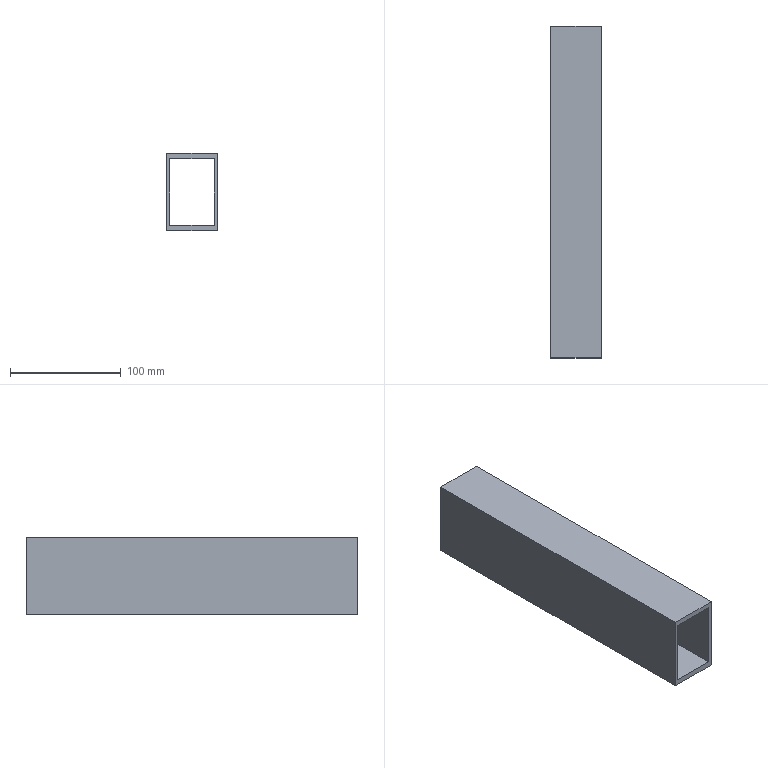Component | SolidWorks | Telescopic2-1 | 1 solid | 10 faces | box 46 x 300 x 70 mm | volume 246000 mm3 | plane 10
build123d program:
from build123d import *

# Parameters (mm, degrees)
SKETCH1_W           = 70
SKETCH1_H           = 46
BOSS_EXTRUDE1_DEPTH = 300
SKETCH2_W           = 60
SKETCH2_H           = 40
CUT_EXTRUDE1_DEPTH  = 303.909


with BuildPart() as part:
    # Sketch1 → Boss-Extrude1 (new body)
    with BuildSketch(Plane.XY):
        Rectangle(SKETCH1_W, SKETCH1_H)
    extrude(amount=BOSS_EXTRUDE1_DEPTH)

    # Sketch2 → Cut-Extrude1 (cut, through all)
    with BuildSketch(Plane.XY.offset(300)):
        Rectangle(SKETCH2_W, SKETCH2_H)
    extrude(amount=-CUT_EXTRUDE1_DEPTH, mode=Mode.SUBTRACT)


solid = part.part

# Placed as in the assembly
solid = solid.moved(Location((-234.371, -793.365, 102.31), (90, 0, 90)))
STEP:
#1=COLOUR_RGB('',0.7922,0.8196,0.9333);
#2=FILL_AREA_STYLE_COLOUR('',#1);
#3=FILL_AREA_STYLE('',(#2));
#4=SURFACE_STYLE_FILL_AREA(#3);
#5=SURFACE_SIDE_STYLE('',(#4));
#6=SURFACE_STYLE_USAGE(.BOTH.,#5);
#7=PRESENTATION_STYLE_ASSIGNMENT((#6));
#8=CARTESIAN_POINT('',(-10.133,-43.046,5.406));
#9=VERTEX_POINT('',#8);
#10=CARTESIAN_POINT('',(-8.322,-43.046,5.406));
#11=VERTEX_POINT('',#10);
#12=CARTESIAN_POINT('',(-10.133,-43.046,5.406));
#13=DIRECTION('',(1.,-0.,0.));
#14=VECTOR('',#13,39.37);
#15=LINE('',#12,#14);
#16=EDGE_CURVE('',#9,#11,#15,.T.);
#17=ORIENTED_EDGE('',*,*,#16,.T.);
#18=CARTESIAN_POINT('',(-8.322,-31.235,5.406));
#19=VERTEX_POINT('',#18);
#20=CARTESIAN_POINT('',(-8.322,-31.235,5.406));
#21=DIRECTION('',(-0.,-1.,0.));
#22=VECTOR('',#21,39.37);
#23=LINE('',#20,#22);
#24=EDGE_CURVE('',#19,#11,#23,.T.);
#25=ORIENTED_EDGE('',*,*,#24,.F.);
#26=CARTESIAN_POINT('',(-10.133,-31.235,5.406));
#27=VERTEX_POINT('',#26);
#28=CARTESIAN_POINT('',(-10.133,-31.235,5.406));
#29=DIRECTION('',(1.,-0.,0.));
#30=VECTOR('',#29,39.37);
#31=LINE('',#28,#30);
#32=EDGE_CURVE('',#27,#19,#31,.T.);
#33=ORIENTED_EDGE('',*,*,#32,.F.);
#34=CARTESIAN_POINT('',(-10.133,-31.235,5.406));
#35=DIRECTION('',(-0.,-1.,0.));
#36=VECTOR('',#35,39.37);
#37=LINE('',#34,#36);
#38=EDGE_CURVE('',#27,#9,#37,.T.);
#39=ORIENTED_EDGE('',*,*,#38,.T.);
#40=EDGE_LOOP('',(#17,#25,#33,#39));
#41=FACE_OUTER_BOUND('',#40,.T.);
#42=CARTESIAN_POINT('',(-10.133,-31.235,5.406));
#43=DIRECTION('',(0.,-0.,-1.));
#44=DIRECTION('',(0.,1.,-0.));
#45=AXIS2_PLACEMENT_3D('',#42,#43,#44);
#46=PLANE('',#45);
#47=ADVANCED_FACE('',(#41),#46,.F.);
#48=CARTESIAN_POINT('',(-8.322,-43.046,2.65));
#49=VERTEX_POINT('',#48);
#50=CARTESIAN_POINT('',(-8.322,-43.046,2.65));
#51=DIRECTION('',(0.,-0.,-1.));
#52=VECTOR('',#51,39.37);
#53=LINE('',#50,#52);
#54=EDGE_CURVE('',#11,#49,#53,.T.);
#55=ORIENTED_EDGE('',*,*,#54,.T.);
#56=CARTESIAN_POINT('',(-8.322,-31.235,2.65));
#57=VERTEX_POINT('',#56);
#58=CARTESIAN_POINT('',(-8.322,-31.235,2.65));
#59=DIRECTION('',(-0.,-1.,0.));
#60=VECTOR('',#59,39.37);
#61=LINE('',#58,#60);
#62=EDGE_CURVE('',#57,#49,#61,.T.);
#63=ORIENTED_EDGE('',*,*,#62,.F.);
#64=CARTESIAN_POINT('',(-8.322,-31.235,2.65));
#65=DIRECTION('',(0.,-0.,-1.));
#66=VECTOR('',#65,39.37);
#67=LINE('',#64,#66);
#68=EDGE_CURVE('',#19,#57,#67,.T.);
#69=ORIENTED_EDGE('',*,*,#68,.F.);
#70=ORIENTED_EDGE('',*,*,#24,.T.);
#71=EDGE_LOOP('',(#55,#63,#69,#70));
#72=FACE_OUTER_BOUND('',#71,.T.);
#73=CARTESIAN_POINT('',(-8.322,-31.235,2.65));
#74=DIRECTION('',(-1.,0.,-0.));
#75=DIRECTION('',(-0.,-1.,0.));
#76=AXIS2_PLACEMENT_3D('',#73,#74,#75);
#77=PLANE('',#76);
#78=ADVANCED_FACE('',(#72),#77,.F.);
#79=CARTESIAN_POINT('',(-10.133,-43.046,2.65));
#80=VERTEX_POINT('',#79);
#81=CARTESIAN_POINT('',(-10.133,-43.046,2.65));
#82=DIRECTION('',(-1.,0.,-0.));
#83=VECTOR('',#82,39.37);
#84=LINE('',#81,#83);
#85=EDGE_CURVE('',#49,#80,#84,.T.);
#86=ORIENTED_EDGE('',*,*,#85,.T.);
#87=CARTESIAN_POINT('',(-10.133,-31.235,2.65));
#88=VERTEX_POINT('',#87);
#89=CARTESIAN_POINT('',(-10.133,-31.235,2.65));
#90=DIRECTION('',(-0.,-1.,0.));
#91=VECTOR('',#90,39.37);
#92=LINE('',#89,#91);
#93=EDGE_CURVE('',#88,#80,#92,.T.);
#94=ORIENTED_EDGE('',*,*,#93,.F.);
#95=CARTESIAN_POINT('',(-10.133,-31.235,2.65));
#96=DIRECTION('',(-1.,0.,-0.));
#97=VECTOR('',#96,39.37);
#98=LINE('',#95,#97);
#99=EDGE_CURVE('',#57,#88,#98,.T.);
#100=ORIENTED_EDGE('',*,*,#99,.F.);
#101=ORIENTED_EDGE('',*,*,#62,.T.);
#102=EDGE_LOOP('',(#86,#94,#100,#101));
#103=FACE_OUTER_BOUND('',#102,.T.);
#104=CARTESIAN_POINT('',(-10.133,-31.235,2.65));
#105=DIRECTION('',(-0.,0.,1.));
#106=DIRECTION('',(-0.,-1.,0.));
#107=AXIS2_PLACEMENT_3D('',#104,#105,#106);
#108=PLANE('',#107);
#109=ADVANCED_FACE('',(#103),#108,.F.);
#110=CARTESIAN_POINT('',(-10.133,-43.046,2.65));
#111=DIRECTION('',(-0.,0.,1.));
#112=VECTOR('',#111,39.37);
#113=LINE('',#110,#112);
#114=EDGE_CURVE('',#80,#9,#113,.T.);
#115=ORIENTED_EDGE('',*,*,#114,.T.);
#116=ORIENTED_EDGE('',*,*,#38,.F.);
#117=CARTESIAN_POINT('',(-10.133,-31.235,2.65));
#118=DIRECTION('',(-0.,0.,1.));
#119=VECTOR('',#118,39.37);
#120=LINE('',#117,#119);
#121=EDGE_CURVE('',#88,#27,#120,.T.);
#122=ORIENTED_EDGE('',*,*,#121,.F.);
#123=ORIENTED_EDGE('',*,*,#93,.T.);
#124=EDGE_LOOP('',(#115,#116,#122,#123));
#125=FACE_OUTER_BOUND('',#124,.T.);
#126=CARTESIAN_POINT('',(-10.133,-31.235,2.65));
#127=DIRECTION('',(1.,-0.,0.));
#128=DIRECTION('',(0.,1.,-0.));
#129=AXIS2_PLACEMENT_3D('',#126,#127,#128);
#130=PLANE('',#129);
#131=ADVANCED_FACE('',(#125),#130,.F.);
#132=CARTESIAN_POINT('',(-8.44,-31.235,5.209));
#133=VERTEX_POINT('',#132);
#134=CARTESIAN_POINT('',(-8.44,-31.235,2.847));
#135=VERTEX_POINT('',#134);
#136=CARTESIAN_POINT('',(-8.44,-31.235,2.847));
#137=DIRECTION('',(0.,-0.,-1.));
#138=VECTOR('',#137,39.37);
#139=LINE('',#136,#138);
#140=EDGE_CURVE('',#133,#135,#139,.T.);
#141=ORIENTED_EDGE('',*,*,#140,.F.);
#142=CARTESIAN_POINT('',(-10.015,-31.235,5.209));
#143=VERTEX_POINT('',#142);
#144=CARTESIAN_POINT('',(-10.015,-31.235,5.209));
#145=DIRECTION('',(1.,-0.,0.));
#146=VECTOR('',#145,39.37);
#147=LINE('',#144,#146);
#148=EDGE_CURVE('',#143,#133,#147,.T.);
#149=ORIENTED_EDGE('',*,*,#148,.F.);
#150=CARTESIAN_POINT('',(-10.015,-31.235,2.847));
#151=VERTEX_POINT('',#150);
#152=CARTESIAN_POINT('',(-10.015,-31.235,2.847));
#153=DIRECTION('',(-0.,0.,1.));
#154=VECTOR('',#153,39.37);
#155=LINE('',#152,#154);
#156=EDGE_CURVE('',#151,#143,#155,.T.);
#157=ORIENTED_EDGE('',*,*,#156,.F.);
#158=CARTESIAN_POINT('',(-10.015,-31.235,2.847));
#159=DIRECTION('',(-1.,0.,-0.));
#160=VECTOR('',#159,39.37);
#161=LINE('',#158,#160);
#162=EDGE_CURVE('',#135,#151,#161,.T.);
#163=ORIENTED_EDGE('',*,*,#162,.F.);
#164=EDGE_LOOP('',(#141,#149,#157,#163));
#165=FACE_BOUND('',#164,.T.);
#166=ORIENTED_EDGE('',*,*,#32,.T.);
#167=ORIENTED_EDGE('',*,*,#68,.T.);
#168=ORIENTED_EDGE('',*,*,#99,.T.);
#169=ORIENTED_EDGE('',*,*,#121,.T.);
#170=EDGE_LOOP('',(#166,#167,#168,#169));
#171=FACE_OUTER_BOUND('',#170,.T.);
#172=CARTESIAN_POINT('',(-9.227,-31.235,4.028));
#173=DIRECTION('',(-0.,-1.,0.));
#174=DIRECTION('',(0.,-0.,-1.));
#175=AXIS2_PLACEMENT_3D('',#172,#173,#174);
#176=PLANE('',#175);
#177=ADVANCED_FACE('',(#165,#171),#176,.F.);
#178=CARTESIAN_POINT('',(-10.015,-43.046,5.209));
#179=VERTEX_POINT('',#178);
#180=CARTESIAN_POINT('',(-8.44,-43.046,5.209));
#181=VERTEX_POINT('',#180);
#182=CARTESIAN_POINT('',(-10.015,-43.046,5.209));
#183=DIRECTION('',(1.,-0.,0.));
#184=VECTOR('',#183,39.37);
#185=LINE('',#182,#184);
#186=EDGE_CURVE('',#179,#181,#185,.T.);
#187=ORIENTED_EDGE('',*,*,#186,.T.);
#188=CARTESIAN_POINT('',(-8.44,-43.046,2.847));
#189=VERTEX_POINT('',#188);
#190=CARTESIAN_POINT('',(-8.44,-43.046,2.847));
#191=DIRECTION('',(0.,-0.,-1.));
#192=VECTOR('',#191,39.37);
#193=LINE('',#190,#192);
#194=EDGE_CURVE('',#181,#189,#193,.T.);
#195=ORIENTED_EDGE('',*,*,#194,.T.);
#196=CARTESIAN_POINT('',(-10.015,-43.046,2.847));
#197=VERTEX_POINT('',#196);
#198=CARTESIAN_POINT('',(-10.015,-43.046,2.847));
#199=DIRECTION('',(-1.,0.,-0.));
#200=VECTOR('',#199,39.37);
#201=LINE('',#198,#200);
#202=EDGE_CURVE('',#189,#197,#201,.T.);
#203=ORIENTED_EDGE('',*,*,#202,.T.);
#204=CARTESIAN_POINT('',(-10.015,-43.046,2.847));
#205=DIRECTION('',(-0.,0.,1.));
#206=VECTOR('',#205,39.37);
#207=LINE('',#204,#206);
#208=EDGE_CURVE('',#197,#179,#207,.T.);
#209=ORIENTED_EDGE('',*,*,#208,.T.);
#210=EDGE_LOOP('',(#187,#195,#203,#209));
#211=FACE_BOUND('',#210,.T.);
#212=ORIENTED_EDGE('',*,*,#16,.F.);
#213=ORIENTED_EDGE('',*,*,#114,.F.);
#214=ORIENTED_EDGE('',*,*,#85,.F.);
#215=ORIENTED_EDGE('',*,*,#54,.F.);
#216=EDGE_LOOP('',(#212,#213,#214,#215));
#217=FACE_OUTER_BOUND('',#216,.T.);
#218=CARTESIAN_POINT('',(-9.227,-43.046,4.028));
#219=DIRECTION('',(-0.,-1.,0.));
#220=DIRECTION('',(0.,-0.,-1.));
#221=AXIS2_PLACEMENT_3D('',#218,#219,#220);
#222=PLANE('',#221);
#223=ADVANCED_FACE('',(#211,#217),#222,.T.);
#224=ORIENTED_EDGE('',*,*,#148,.T.);
#225=CARTESIAN_POINT('',(-8.44,-43.046,5.209));
#226=DIRECTION('',(0.,1.,-0.));
#227=VECTOR('',#226,39.37);
#228=LINE('',#225,#227);
#229=EDGE_CURVE('',#181,#133,#228,.T.);
#230=ORIENTED_EDGE('',*,*,#229,.F.);
#231=ORIENTED_EDGE('',*,*,#186,.F.);
#232=CARTESIAN_POINT('',(-10.015,-43.046,5.209));
#233=DIRECTION('',(0.,1.,-0.));
#234=VECTOR('',#233,39.37);
#235=LINE('',#232,#234);
#236=EDGE_CURVE('',#179,#143,#235,.T.);
#237=ORIENTED_EDGE('',*,*,#236,.T.);
#238=EDGE_LOOP('',(#224,#230,#231,#237));
#239=FACE_OUTER_BOUND('',#238,.T.);
#240=CARTESIAN_POINT('',(-10.015,-43.046,5.209));
#241=DIRECTION('',(-0.,0.,1.));
#242=DIRECTION('',(-0.,-1.,0.));
#243=AXIS2_PLACEMENT_3D('',#240,#241,#242);
#244=PLANE('',#243);
#245=ADVANCED_FACE('',(#239),#244,.F.);
#246=ORIENTED_EDGE('',*,*,#156,.T.);
#247=ORIENTED_EDGE('',*,*,#236,.F.);
#248=ORIENTED_EDGE('',*,*,#208,.F.);
#249=CARTESIAN_POINT('',(-10.015,-43.046,2.847));
#250=DIRECTION('',(0.,1.,-0.));
#251=VECTOR('',#250,39.37);
#252=LINE('',#249,#251);
#253=EDGE_CURVE('',#197,#151,#252,.T.);
#254=ORIENTED_EDGE('',*,*,#253,.T.);
#255=EDGE_LOOP('',(#246,#247,#248,#254));
#256=FACE_OUTER_BOUND('',#255,.T.);
#257=CARTESIAN_POINT('',(-10.015,-43.046,2.847));
#258=DIRECTION('',(-1.,0.,-0.));
#259=DIRECTION('',(-0.,-1.,0.));
#260=AXIS2_PLACEMENT_3D('',#257,#258,#259);
#261=PLANE('',#260);
#262=ADVANCED_FACE('',(#256),#261,.F.);
#263=ORIENTED_EDGE('',*,*,#162,.T.);
#264=ORIENTED_EDGE('',*,*,#253,.F.);
#265=ORIENTED_EDGE('',*,*,#202,.F.);
#266=CARTESIAN_POINT('',(-8.44,-43.046,2.847));
#267=DIRECTION('',(0.,1.,-0.));
#268=VECTOR('',#267,39.37);
#269=LINE('',#266,#268);
#270=EDGE_CURVE('',#189,#135,#269,.T.);
#271=ORIENTED_EDGE('',*,*,#270,.T.);
#272=EDGE_LOOP('',(#263,#264,#265,#271));
#273=FACE_OUTER_BOUND('',#272,.T.);
#274=CARTESIAN_POINT('',(-10.015,-43.046,2.847));
#275=DIRECTION('',(0.,-0.,-1.));
#276=DIRECTION('',(0.,1.,-0.));
#277=AXIS2_PLACEMENT_3D('',#274,#275,#276);
#278=PLANE('',#277);
#279=ADVANCED_FACE('',(#273),#278,.F.);
#280=ORIENTED_EDGE('',*,*,#140,.T.);
#281=ORIENTED_EDGE('',*,*,#270,.F.);
#282=ORIENTED_EDGE('',*,*,#194,.F.);
#283=ORIENTED_EDGE('',*,*,#229,.T.);
#284=EDGE_LOOP('',(#280,#281,#282,#283));
#285=FACE_OUTER_BOUND('',#284,.T.);
#286=CARTESIAN_POINT('',(-8.44,-43.046,2.847));
#287=DIRECTION('',(1.,-0.,0.));
#288=DIRECTION('',(0.,1.,-0.));
#289=AXIS2_PLACEMENT_3D('',#286,#287,#288);
#290=PLANE('',#289);
#291=ADVANCED_FACE('',(#285),#290,.F.);
#292=CLOSED_SHELL('',(#47,#78,#109,#131,#177,#223,#245,#262,#279,#291));
#293=MANIFOLD_SOLID_BREP('',#292);
#294=STYLED_ITEM('',(#7),#293);
#295=PRESENTATION_LAYER_ASSIGNMENT('','',(#294));
#296=(LENGTH_UNIT()NAMED_UNIT(*)SI_UNIT($,.METRE.));
#297=LENGTH_MEASURE_WITH_UNIT(LENGTH_MEASURE(0.0254),#296);
#298=DIMENSIONAL_EXPONENTS(1.,0.,0.,0.,0.,0.,0.);
#299=(CONVERSION_BASED_UNIT('',#297)LENGTH_UNIT()NAMED_UNIT(#298));
#300=UNCERTAINTY_MEASURE_WITH_UNIT(LENGTH_MEASURE(0.00001),#299,'','');
#301=(NAMED_UNIT(*)PLANE_ANGLE_UNIT()SI_UNIT($,.RADIAN.));
#302=(NAMED_UNIT(*)SI_UNIT($,.STERADIAN.)SOLID_ANGLE_UNIT());
#303=(GEOMETRIC_REPRESENTATION_CONTEXT(3)GLOBAL_UNCERTAINTY_ASSIGNED_CONTEXT((#300))GLOBAL_UNIT_ASSIGNED_CONTEXT((#299,#301,#302))REPRESENTATION_CONTEXT('',''));
#304=MECHANICAL_DESIGN_GEOMETRIC_PRESENTATION_REPRESENTATION('',(#294),#303);
#305=CARTESIAN_POINT('',(0.,0.,0.));
#306=DIRECTION('',(0.,0.,1.));
#307=DIRECTION('',(1.,0.,0.));
#308=AXIS2_PLACEMENT_3D('',#305,#306,#307);
#309=(LENGTH_UNIT()NAMED_UNIT(*)SI_UNIT($,.METRE.));
#310=LENGTH_MEASURE_WITH_UNIT(LENGTH_MEASURE(0.0254),#309);
#311=DIMENSIONAL_EXPONENTS(1.,0.,0.,0.,0.,0.,0.);
#312=(CONVERSION_BASED_UNIT('',#310)LENGTH_UNIT()NAMED_UNIT(#311));
#313=UNCERTAINTY_MEASURE_WITH_UNIT(LENGTH_MEASURE(0.00001),#312,'','');
#314=(NAMED_UNIT(*)PLANE_ANGLE_UNIT()SI_UNIT($,.RADIAN.));
#315=(NAMED_UNIT(*)SI_UNIT($,.STERADIAN.)SOLID_ANGLE_UNIT());
#316=(GEOMETRIC_REPRESENTATION_CONTEXT(3)GLOBAL_UNCERTAINTY_ASSIGNED_CONTEXT((#313))GLOBAL_UNIT_ASSIGNED_CONTEXT((#312,#314,#315))REPRESENTATION_CONTEXT('',''));
#317=ADVANCED_BREP_SHAPE_REPRESENTATION('',(#293,#308),#316);